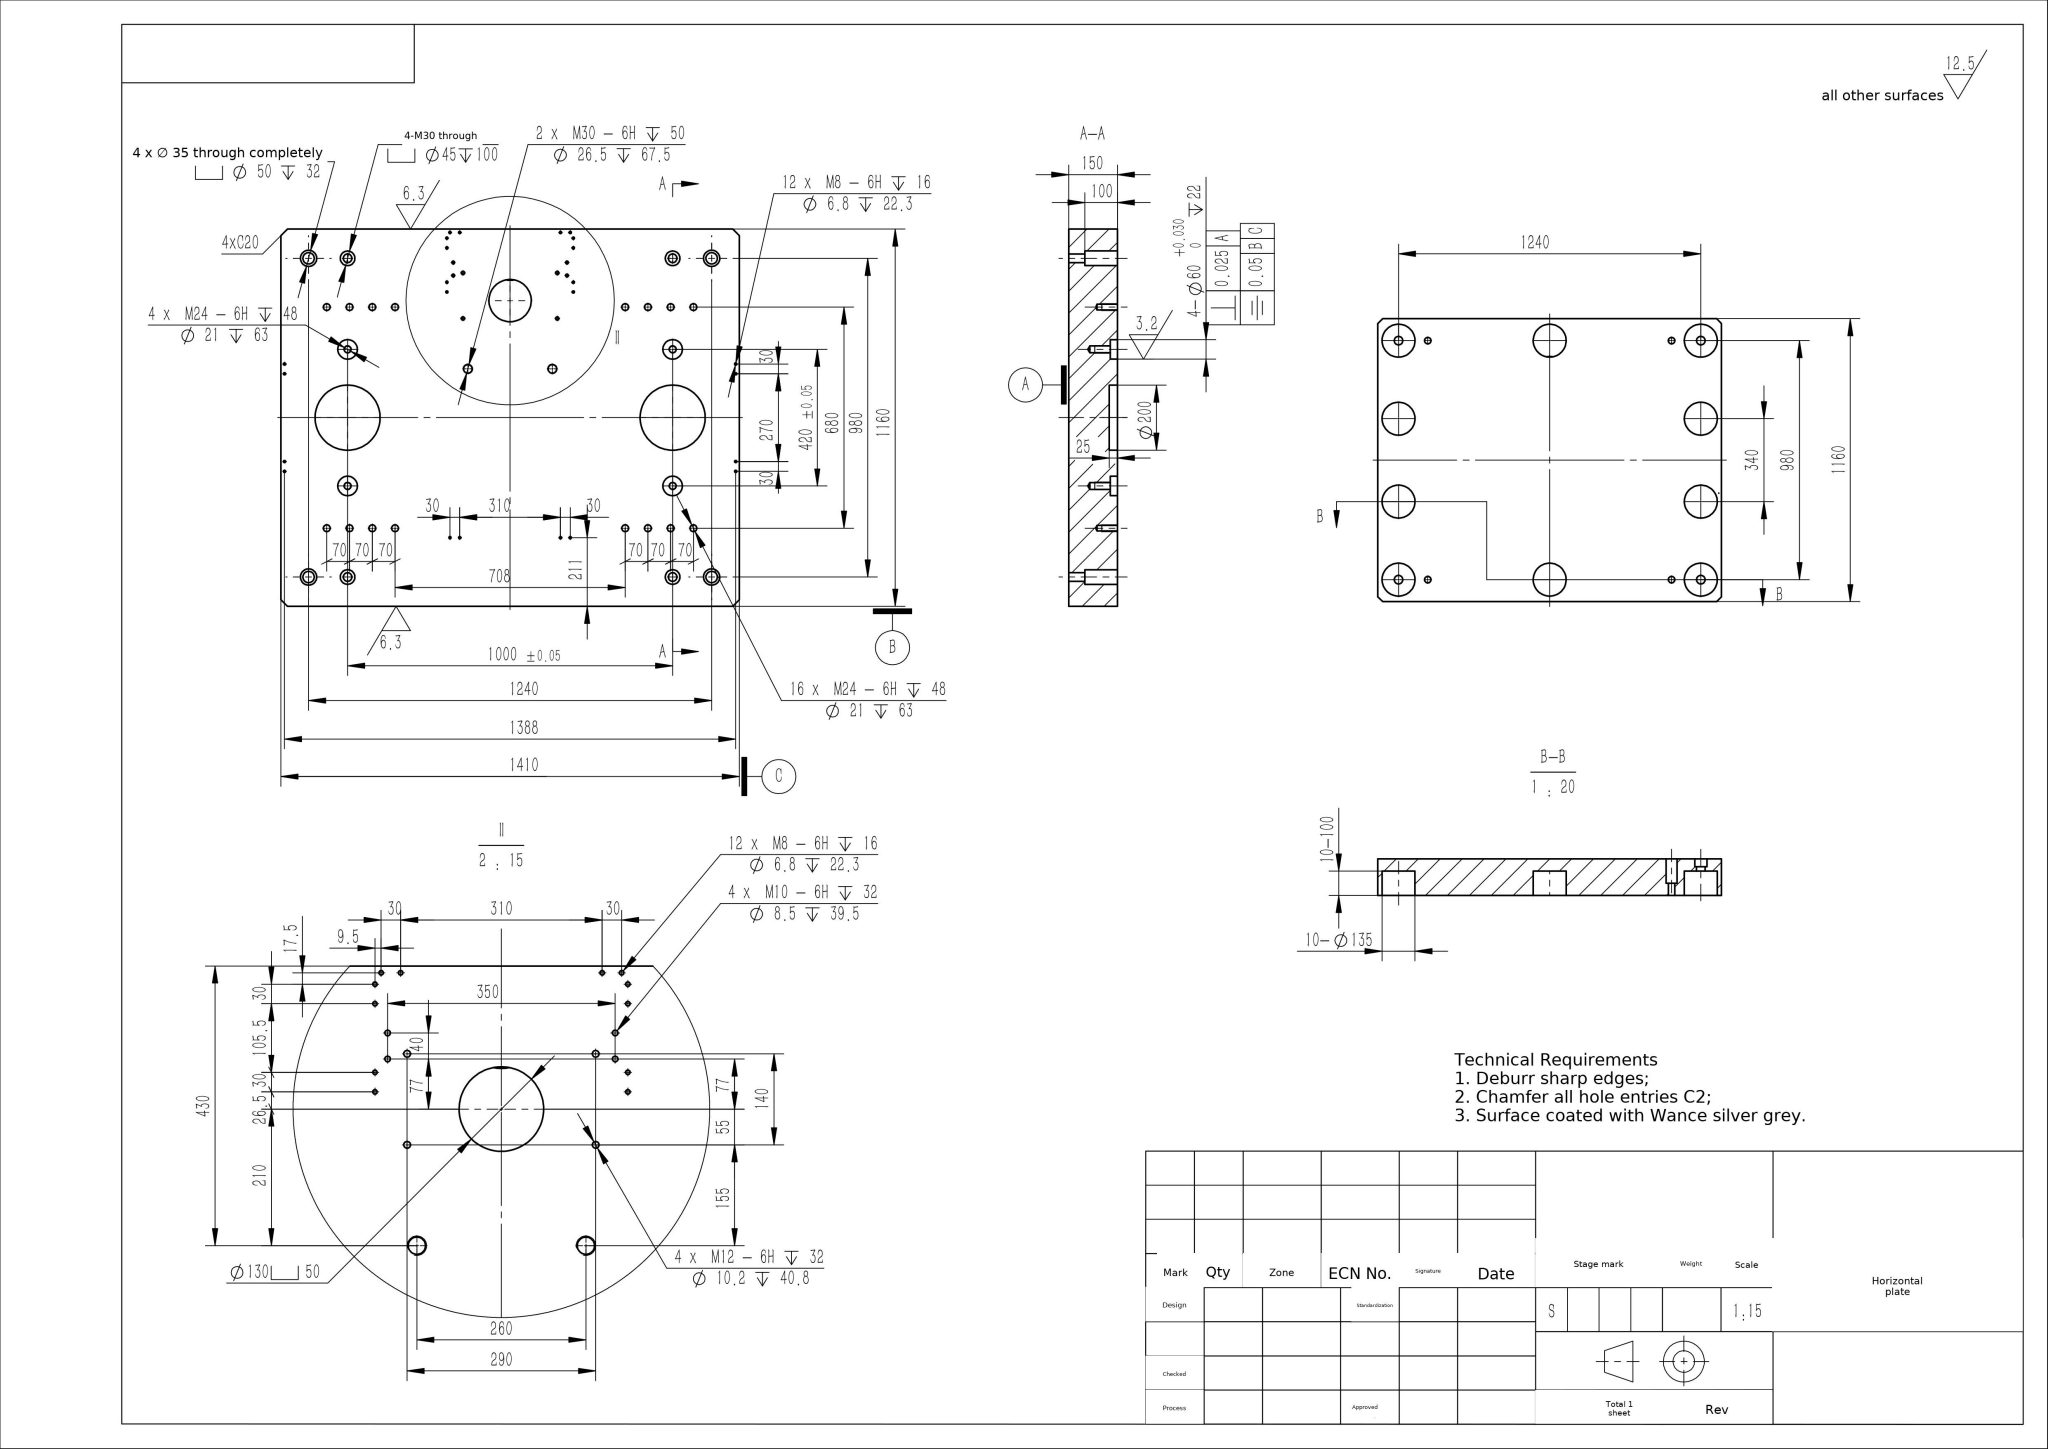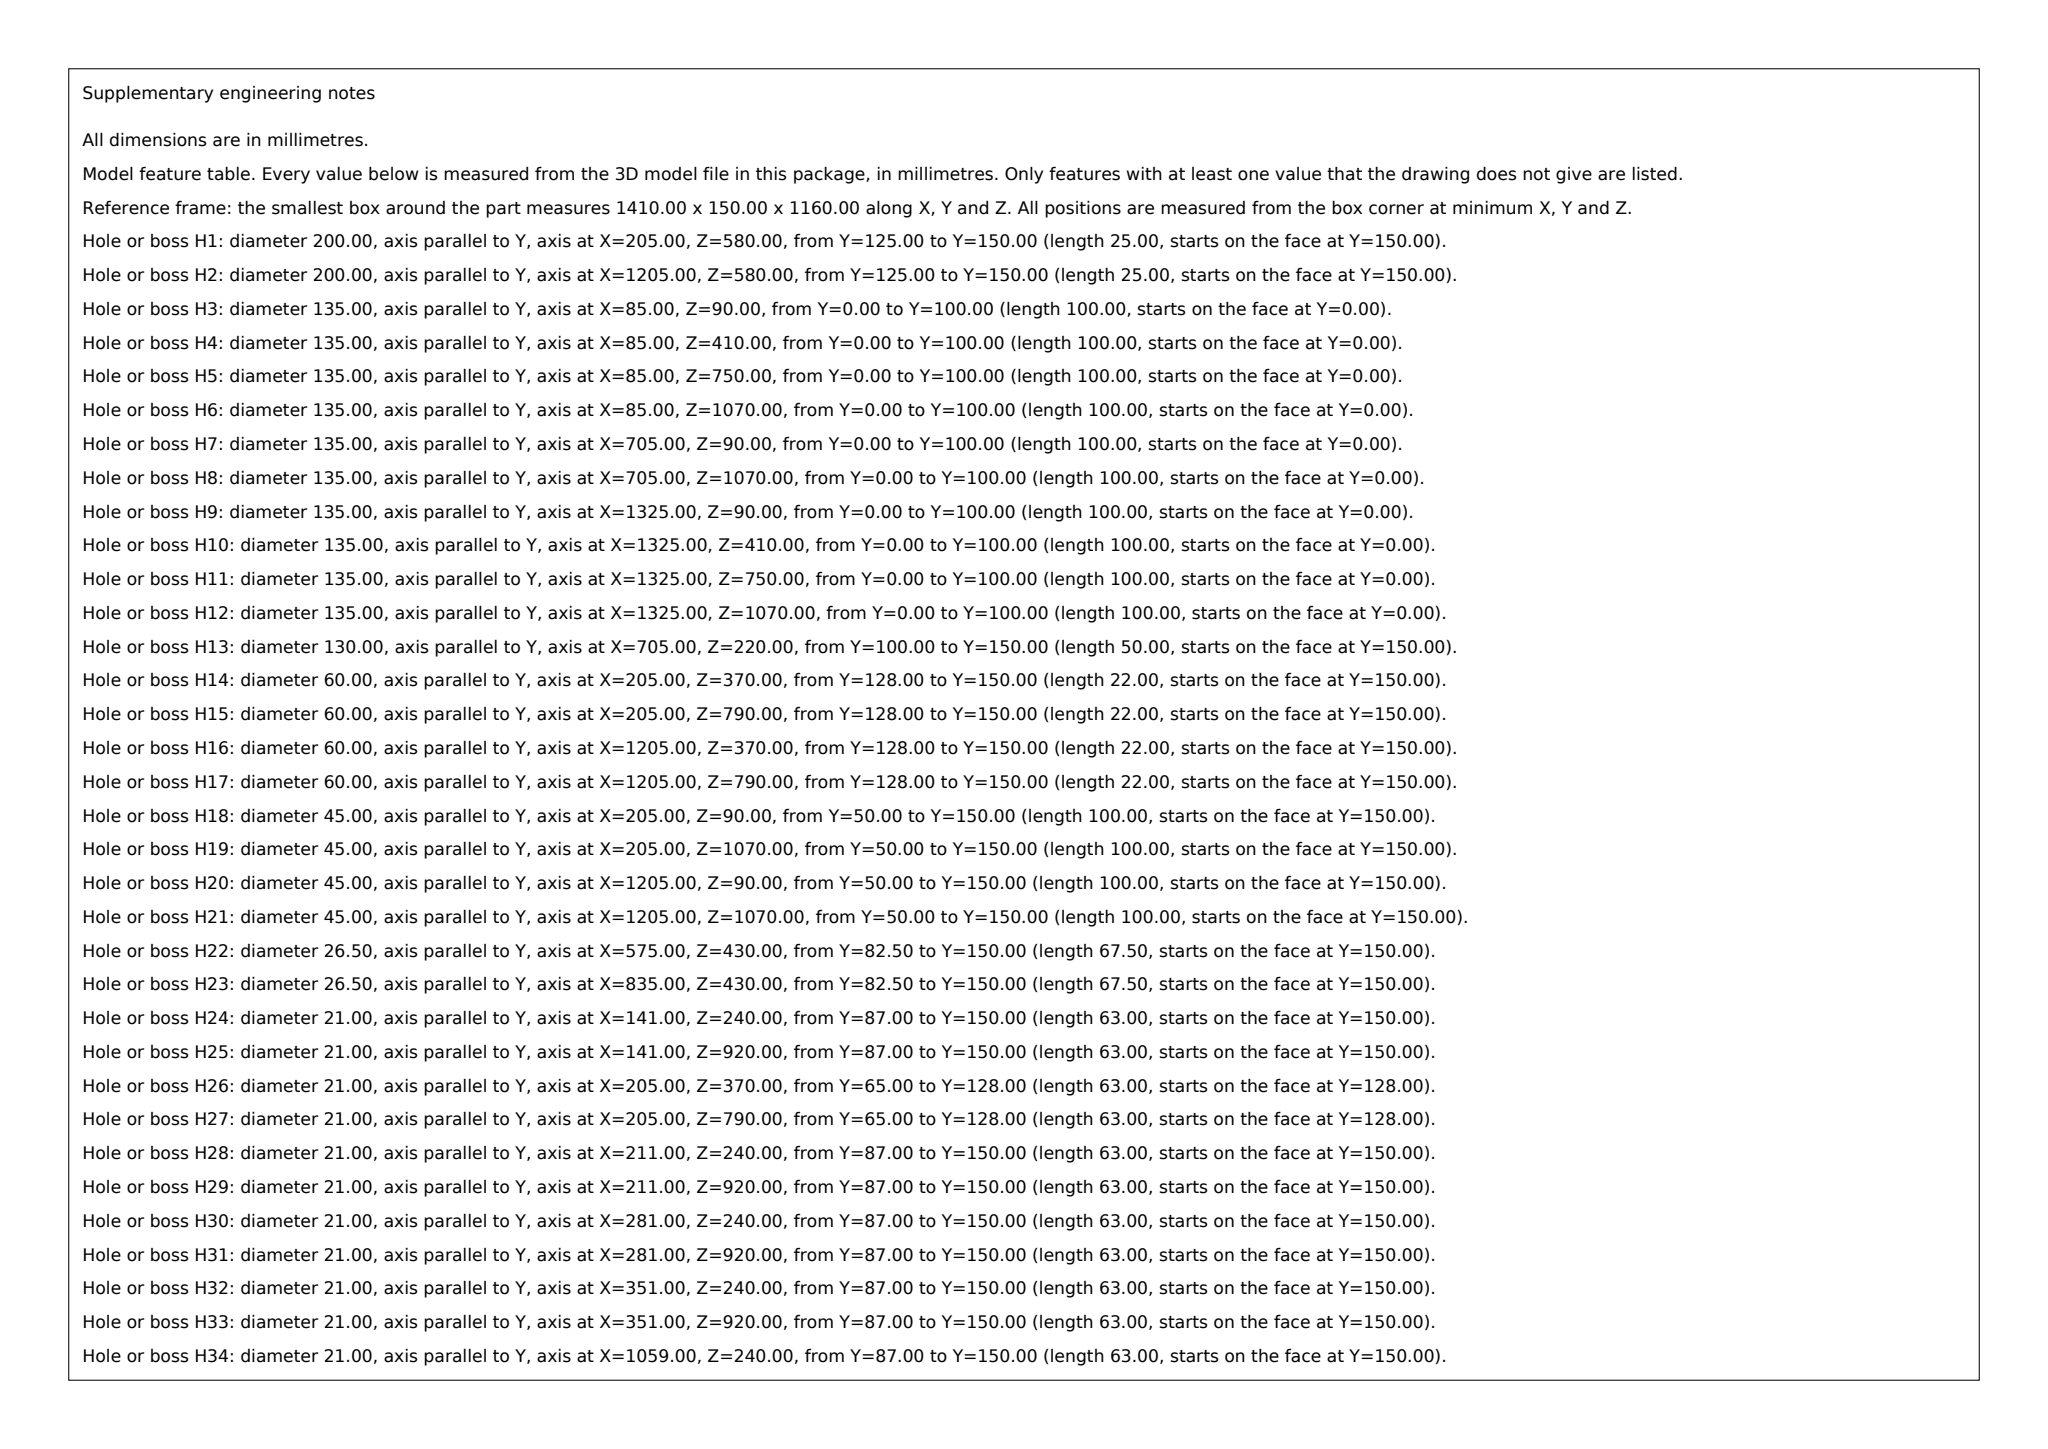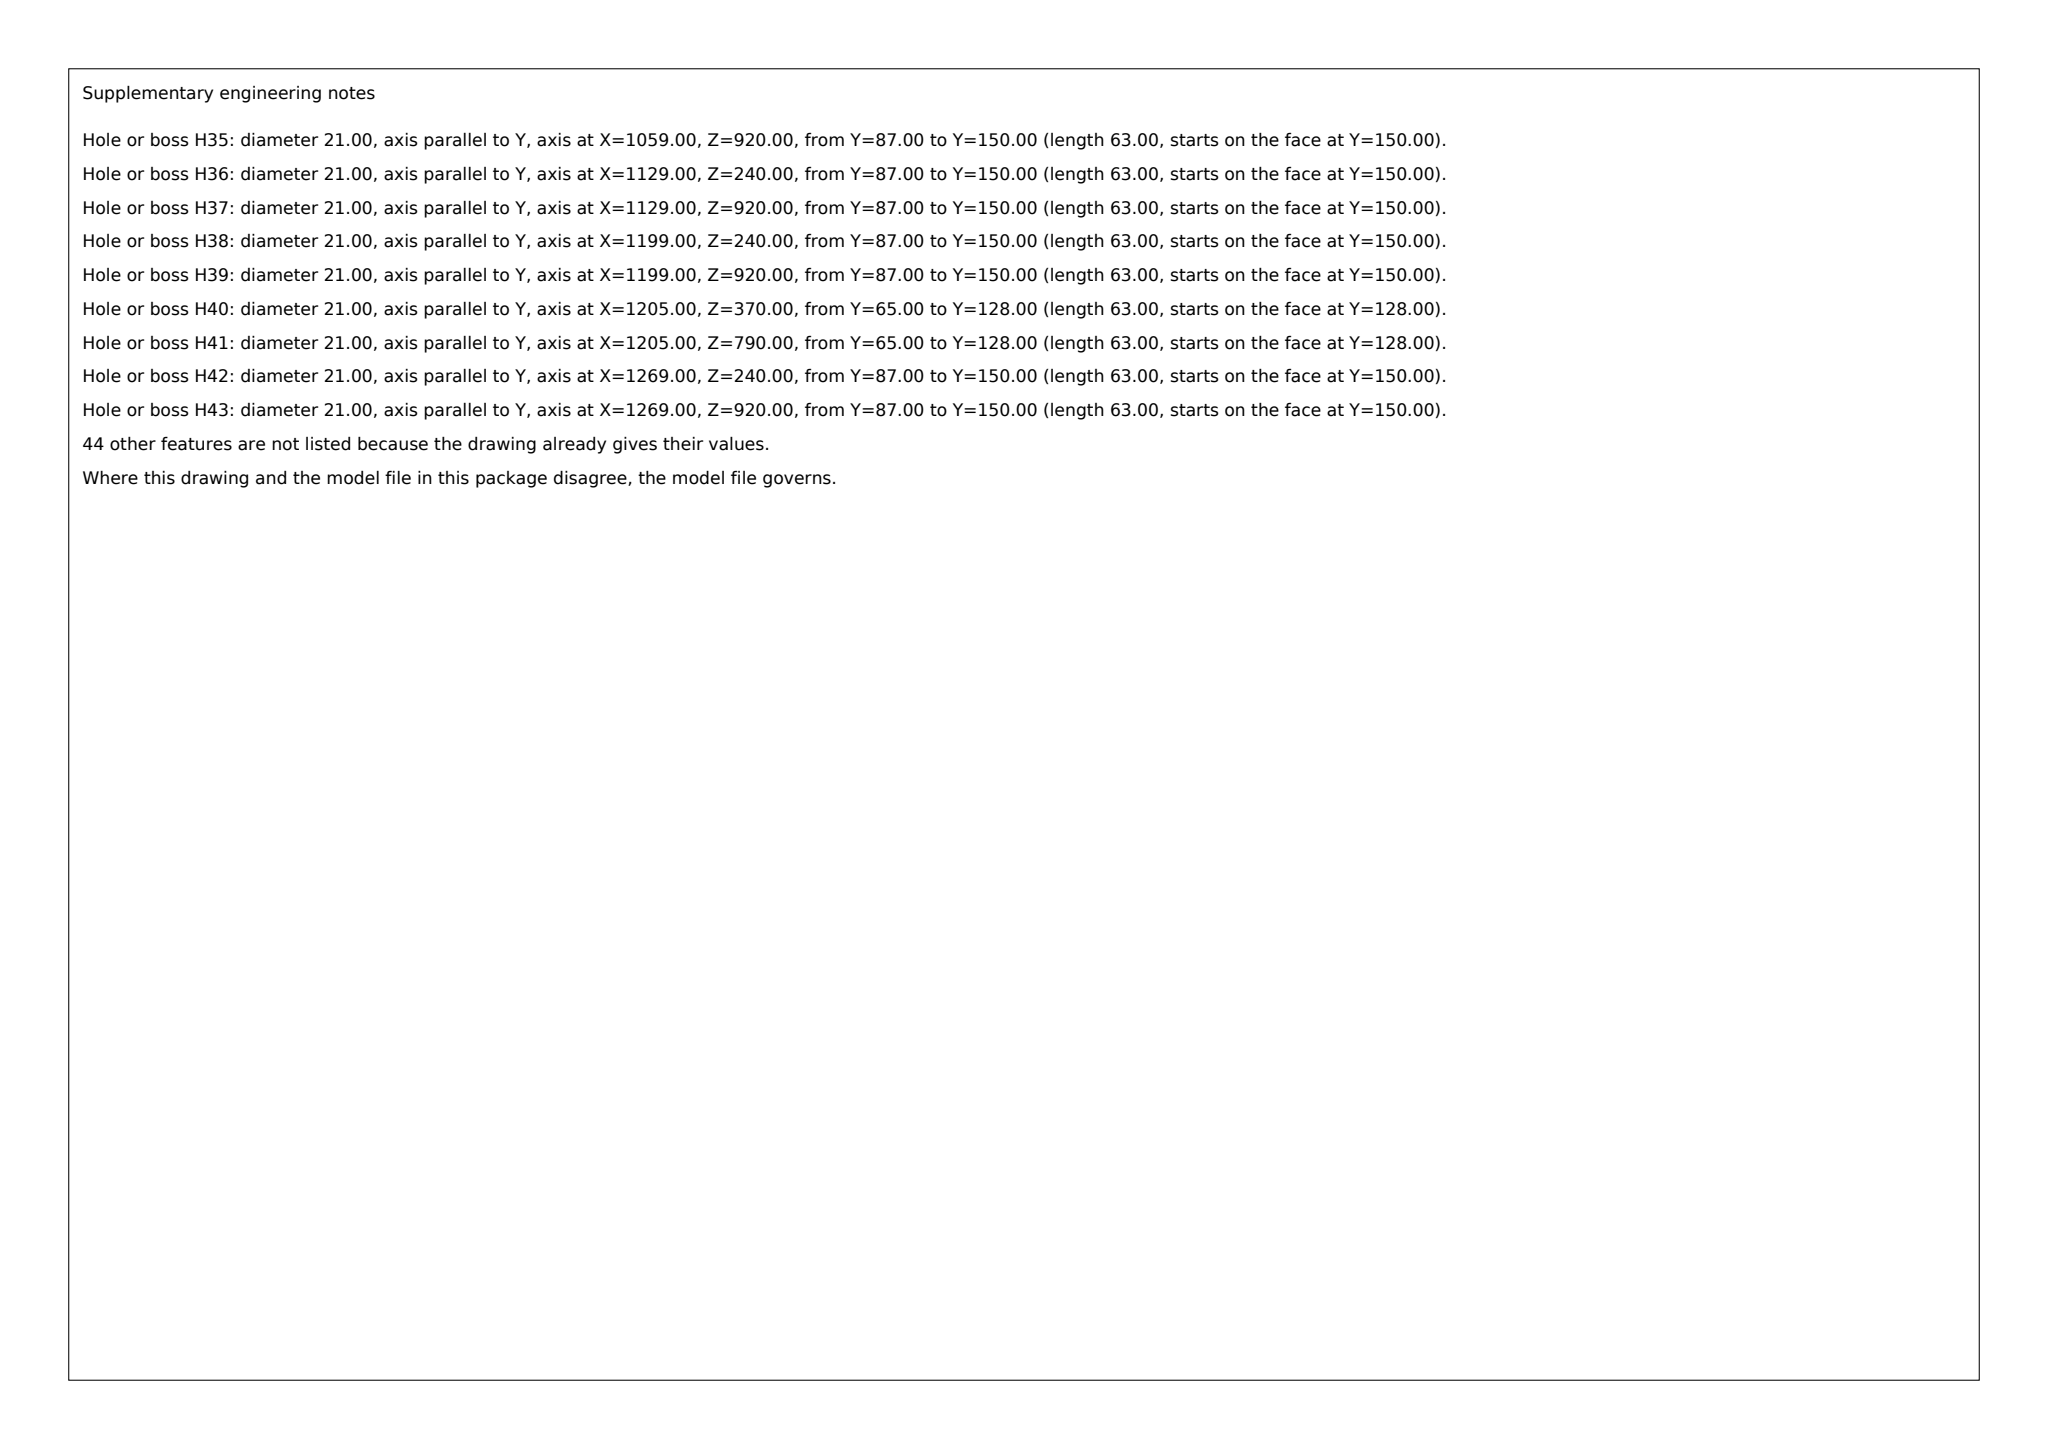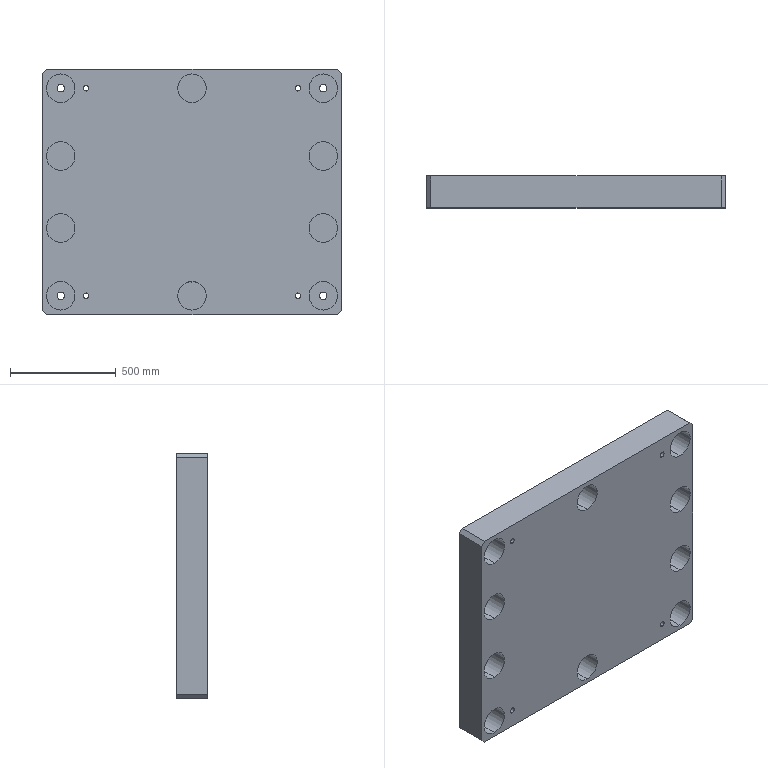Part | SolidWorks | mm | 1 solid | 317 faces | box 1410 x 150 x 1160 mm | volume 226784598 mm3 | cylinder 174 | cone 108 | plane 35 | commonest cylinder face diameters 6.8 x48 21 x40 135 x20 26.5 x12 45 x8 50 x8 35 x8 8.5 x8
build123d program:
from build123d import *

# Parameters (mm, degrees)
SKETCH2_W                                          = 1410
SKETCH2_H                                          = 720
BOSS_EXTRUDE1_DEPTH                                = 150
SKETCH4_R                                          = 100
CUT_EXTRUDE1_DEPTH                                 = 25
SKETCH6_R                                          = 30
CUT_EXTRUDE3_DEPTH                                 = 22
SKETCH24_W                                         = 1410
SKETCH24_H                                         = 150
BOSS_EXTRUDE5_DEPTH                                = 220
M12_TAPPED_HOLE1_D                                 = 10.2
M12_TAPPED_HOLE1_DEPTH                             = 40.75
M12_TAPPED_HOLE1_TIP                               = 3.064
SKETCH28_R                                         = 65
CUT_EXTRUDE8_DEPTH                                 = 50
SKETCH41_W                                         = 1410
SKETCH41_H                                         = 150
CUT_EXTRUDE11_DEPTH                                = 1
M30_TAPPED_HOLE1_D                                 = 26.5
M30_TAPPED_HOLE1_DEPTH                             = 67.5
M30_TAPPED_HOLE1_TIP                               = 7.961
M10_TAPPED_HOLE2_D                                 = 8.5
M10_TAPPED_HOLE2_DEPTH                             = 39.5
M10_TAPPED_HOLE2_TIP                               = 2.554
SKETCH60_W                                         = 1410
SKETCH60_H                                         = 150
BOSS_EXTRUDE7_DEPTH                                = 24
SKETCH67_W                                         = 1410
SKETCH67_H                                         = 150
BOSS_EXTRUDE9_DEPTH                                = 197
M24_TAPPED_HOLE1_AT_2_COUNT                        = 2
M24_TAPPED_HOLE1_AT_2_PITCH                        = 70
M24_TAPPED_HOLE1_AT_3_COUNT                        = 2
M24_TAPPED_HOLE1_AT_3_PITCH                        = 140
M24_TAPPED_HOLE1_AT_4_COUNT                        = 2
M24_TAPPED_HOLE1_AT_4_PITCH                        = 210
SKETCH73_R                                         = 67.5
CUT_EXTRUDE15_DEPTH                                = 100
HOLE_SIZE_ACCORDING_TO_TYPE_1_OF_HEXAG_D           = 35
HOLE_SIZE_ACCORDING_TO_TYPE_1_OF_HEXAG_CBORE_D     = 50
HOLE_SIZE_ACCORDING_TO_TYPE_1_OF_HEXAG_CBORE_DEPTH = 32
HOLE_SIZE_ACCORDING_TO_TYPE_1_OF_H_2_D             = 35
HOLE_SIZE_ACCORDING_TO_TYPE_1_OF_H_2_CBORE_D       = 50
HOLE_SIZE_ACCORDING_TO_TYPE_1_OF_H_2_CBORE_DEPTH   = 32
M30_TAPPED_HOLE2_D                                 = 26.5
SKETCH77_R                                         = 22.5
CUT_EXTRUDE16_DEPTH                                = 100
M8_TAPPED_HOLE1_D                                  = 6.8
M8_TAPPED_HOLE1_DEPTH                              = 22.25
M8_TAPPED_HOLE1_TIP                                = 2.043
M24_TAPPED_HOLE2_D                                 = 21
M24_TAPPED_HOLE2_DEPTH                             = 63
M24_TAPPED_HOLE2_TIP                               = 6.309
CHAMFER1_SIZE                                      = 20


with BuildPart() as part:
    # Sketch2 → Boss-Extrude1 (new body)
    with BuildSketch(Plane(origin=(0, 0, 0), x_dir=(1, 0, 0), z_dir=(0, 1, 0))):
        Rectangle(SKETCH2_W, SKETCH2_H)
    extrude(amount=-BOSS_EXTRUDE1_DEPTH)

    # Sketch4 → Cut-Extrude1 (cut)
    with BuildSketch(Plane(origin=(0, 0, 0), x_dir=(-1, 0, 0), z_dir=(0, 1, 0))):
        with Locations(Location((-500, 0, 0), (0, 0, 90))):
            Circle(SKETCH4_R)
        with Locations(Location((500, 0, 0), (0, 0, 90))):
            Circle(SKETCH4_R)
    extrude(amount=-CUT_EXTRUDE1_DEPTH, mode=Mode.SUBTRACT)

    # Sketch6 → Cut-Extrude3 (cut)
    with BuildSketch(Plane(origin=(0, 0, 0), x_dir=(-1, 0, 0), z_dir=(0, 1, 0))):
        with Locations(Location((-500, 210, 0), (0, 0, 90))):
            Circle(SKETCH6_R)
        with Locations(Location((500, 210, 0), (0, 0, 90))):
            Circle(SKETCH6_R)
        with Locations(Location((500, -210, 0), (0, 0, 90))):
            Circle(SKETCH6_R)
        with Locations(Location((-500, -210, 0), (0, 0, 90))):
            Circle(SKETCH6_R)
    extrude(amount=-CUT_EXTRUDE3_DEPTH, mode=Mode.SUBTRACT)

    # Sketch24 → Boss-Extrude5 (add)
    with BuildSketch(Plane(origin=(0, 0, -360), x_dir=(-1, 0, 0), z_dir=(0, 0, -1))):
        with Locations((0, -75)):
            Rectangle(SKETCH24_W, SKETCH24_H)
    extrude(amount=BOSS_EXTRUDE5_DEPTH)

    # M12 Tapped Hole1
    with Locations(Plane(origin=(0, 0, 0), x_dir=(1, 0, 0), z_dir=(0, 1, 0))):
        with Locations((145, 305), (145, 445), (-145, 305), (-145, 445)):
            Hole(M12_TAPPED_HOLE1_D / 2, depth=M12_TAPPED_HOLE1_DEPTH)
            with Locations((0, 0, -(M12_TAPPED_HOLE1_DEPTH + M12_TAPPED_HOLE1_TIP / 2))):  # 118° drill point
                Cone(0, M12_TAPPED_HOLE1_D / 2, M12_TAPPED_HOLE1_TIP, mode=Mode.SUBTRACT)

    # Sketch28 → Cut-Extrude8 (cut)
    with BuildSketch(Plane(origin=(0, 0, 0), x_dir=(-1, 0, 0), z_dir=(0, 1, 0))):
        with Locations(Location((0, -360, 0), (0, 0, 90))):
            Circle(SKETCH28_R)
    extrude(amount=-CUT_EXTRUDE8_DEPTH, mode=Mode.SUBTRACT)

    # Sketch41 → Cut-Extrude11 (cut)
    with BuildSketch(Plane.XY.offset(360)):
        with Locations((0, -75)):
            Rectangle(SKETCH41_W, SKETCH41_H)
    extrude(amount=-CUT_EXTRUDE11_DEPTH, mode=Mode.SUBTRACT)

    # M30 Tapped Hole1
    with Locations(Plane(origin=(0, 0, 0), x_dir=(1, 0, 0), z_dir=(0, 1, 0))):
        with Locations((130, 150), (-130, 150)):
            Hole(M30_TAPPED_HOLE1_D / 2, depth=M30_TAPPED_HOLE1_DEPTH)
            with Locations((0, 0, -(M30_TAPPED_HOLE1_DEPTH + M30_TAPPED_HOLE1_TIP / 2))):  # 118° drill point
                Cone(0, M30_TAPPED_HOLE1_D / 2, M30_TAPPED_HOLE1_TIP, mode=Mode.SUBTRACT)

    # M10 Tapped Hole2
    with Locations(Plane(origin=(0, 0, 0), x_dir=(1, 0, 0), z_dir=(0, 1, 0))):
        with Locations((175, 477), (175, 437), (-175, 477), (-175, 437)):
            Hole(M10_TAPPED_HOLE2_D / 2, depth=M10_TAPPED_HOLE2_DEPTH)
            with Locations((0, 0, -(M10_TAPPED_HOLE2_DEPTH + M10_TAPPED_HOLE2_TIP / 2))):  # 118° drill point
                Cone(0, M10_TAPPED_HOLE2_D / 2, M10_TAPPED_HOLE2_TIP, mode=Mode.SUBTRACT)

    # Sketch60 → Boss-Extrude7 (add)
    with BuildSketch(Plane.XY.offset(359)):
        with Locations((0, -75)):
            Rectangle(SKETCH60_W, SKETCH60_H)
    extrude(amount=BOSS_EXTRUDE7_DEPTH)

    # Sketch67 → Boss-Extrude9 (add)
    with BuildSketch(Plane.XY.offset(383)):
        with Locations((0, -75)):
            Rectangle(SKETCH67_W, SKETCH67_H)
    extrude(amount=BOSS_EXTRUDE9_DEPTH)

    # Sketch71 → M24 Tapped Hole1 (revolve, cut)
    with BuildSketch(Plane(origin=(354, 0, -340), x_dir=(0, 0, 1), z_dir=(1, 0, 0))):
        Polygon((0, 0), (0, 69.309), (10.5, 63), (10.5, 0), align=None)
    m24_tapped_hole1 = revolve(axis=Axis((354, 6.35, -340), (0, -1, 0)), mode=Mode.SUBTRACT)

    # M24 Tapped Hole1 at 2: M24 Tapped Hole1 ×2
    with Locations(*[(i * M24_TAPPED_HOLE1_AT_2_PITCH, 0, 0) for i in range(1, M24_TAPPED_HOLE1_AT_2_COUNT)]):
        add(m24_tapped_hole1, mode=Mode.SUBTRACT)

    # M24 Tapped Hole1 at 3: M24 Tapped Hole1 ×2
    with Locations(*[(i * M24_TAPPED_HOLE1_AT_3_PITCH, 0, 0) for i in range(1, M24_TAPPED_HOLE1_AT_3_COUNT)]):
        add(m24_tapped_hole1, mode=Mode.SUBTRACT)

    # M24 Tapped Hole1 at 4: M24 Tapped Hole1 ×2
    with Locations(*[(i * M24_TAPPED_HOLE1_AT_4_PITCH, 0, 0) for i in range(1, M24_TAPPED_HOLE1_AT_4_COUNT)]):
        add(m24_tapped_hole1, mode=Mode.SUBTRACT)

    # Mirror11: M24 Tapped Hole1 across plane
    add(m24_tapped_hole1.mirror(Plane(origin=(0, 0, 0), x_dir=(0, 0, 1), z_dir=(1, 0, 0))), mode=Mode.SUBTRACT)

    # Mirror11 copy 1 sketch → Mirror11 copy 1 (revolve, cut)
    with BuildSketch(Plane(origin=(-424, 0, -340), x_dir=(0, 0, 1), z_dir=(-1, 0, 0))):
        Polygon((0, 0), (0, -69.309), (10.5, -63), (10.5, 0), align=None)
    revolve(axis=Axis((-424, 6.35, -340), (0, 1, 0)), mode=Mode.SUBTRACT)

    # Mirror11 copy 2 sketch → Mirror11 copy 2 (revolve, cut)
    with BuildSketch(Plane(origin=(-494, 0, -340), x_dir=(0, 0, 1), z_dir=(-1, 0, 0))):
        Polygon((0, 0), (0, -69.309), (10.5, -63), (10.5, 0), align=None)
    revolve(axis=Axis((-494, 6.35, -340), (0, 1, 0)), mode=Mode.SUBTRACT)

    # Mirror11 copy 3 sketch → Mirror11 copy 3 (revolve, cut)
    with BuildSketch(Plane(origin=(-564, 0, -340), x_dir=(0, 0, 1), z_dir=(-1, 0, 0))):
        Polygon((0, 0), (0, -69.309), (10.5, -63), (10.5, 0), align=None)
    revolve(axis=Axis((-564, 6.35, -340), (0, 1, 0)), mode=Mode.SUBTRACT)

    # Mirror12: M24 Tapped Hole1 across plane
    add(m24_tapped_hole1.mirror(Plane.XY), mode=Mode.SUBTRACT)

    # Mirror12 copy 1 sketch → Mirror12 copy 1 (revolve, cut)
    with BuildSketch(Plane(origin=(424, 0, 340), x_dir=(0, 0, -1), z_dir=(1, 0, 0))):
        Polygon((0, 0), (0, -69.309), (10.5, -63), (10.5, 0), align=None)
    revolve(axis=Axis((424, 6.35, 340), (0, 1, 0)), mode=Mode.SUBTRACT)

    # Mirror12 copy 2 sketch → Mirror12 copy 2 (revolve, cut)
    with BuildSketch(Plane(origin=(494, 0, 340), x_dir=(0, 0, -1), z_dir=(1, 0, 0))):
        Polygon((0, 0), (0, -69.309), (10.5, -63), (10.5, 0), align=None)
    revolve(axis=Axis((494, 6.35, 340), (0, 1, 0)), mode=Mode.SUBTRACT)

    # Mirror12 copy 3 sketch → Mirror12 copy 3 (revolve, cut)
    with BuildSketch(Plane(origin=(564, 0, 340), x_dir=(0, 0, -1), z_dir=(1, 0, 0))):
        Polygon((0, 0), (0, -69.309), (10.5, -63), (10.5, 0), align=None)
    revolve(axis=Axis((564, 6.35, 340), (0, 1, 0)), mode=Mode.SUBTRACT)

    # Mirror12 copy 4 sketch → Mirror12 copy 4 (revolve, cut)
    with BuildSketch(Plane(origin=(-354, 0, 340), x_dir=(0, 0, -1), z_dir=(-1, 0, 0))):
        Polygon((0, 0), (0, 69.309), (10.5, 63), (10.5, 0), align=None)
    revolve(axis=Axis((-354, 6.35, 340), (0, -1, 0)), mode=Mode.SUBTRACT)

    # Mirror12 copy 5 sketch → Mirror12 copy 5 (revolve, cut)
    with BuildSketch(Plane(origin=(-424, 0, 340), x_dir=(0, 0, -1), z_dir=(-1, 0, 0))):
        Polygon((0, 0), (0, 69.309), (10.5, 63), (10.5, 0), align=None)
    revolve(axis=Axis((-424, 6.35, 340), (0, -1, 0)), mode=Mode.SUBTRACT)

    # Mirror12 copy 6 sketch → Mirror12 copy 6 (revolve, cut)
    with BuildSketch(Plane(origin=(-494, 0, 340), x_dir=(0, 0, -1), z_dir=(-1, 0, 0))):
        Polygon((0, 0), (0, 69.309), (10.5, 63), (10.5, 0), align=None)
    revolve(axis=Axis((-494, 6.35, 340), (0, -1, 0)), mode=Mode.SUBTRACT)

    # Mirror12 copy 7 sketch → Mirror12 copy 7 (revolve, cut)
    with BuildSketch(Plane(origin=(-564, 0, 340), x_dir=(0, 0, -1), z_dir=(-1, 0, 0))):
        Polygon((0, 0), (0, 69.309), (10.5, 63), (10.5, 0), align=None)
    revolve(axis=Axis((-564, 6.35, 340), (0, -1, 0)), mode=Mode.SUBTRACT)

    # Sketch73 → Cut-Extrude15 (cut)
    with BuildSketch(Plane(origin=(0, -150, 0), x_dir=(-1, 0, 0), z_dir=(0, -1, 0))):
        with Locations(Location((-620, 490, 0), (0, 0, 90))):
            Circle(SKETCH73_R)
        with Locations(Location((-620, -490, 0), (0, 0, 90))):
            Circle(SKETCH73_R)
        with Locations(Location((0, 490, 0), (0, 0, 90))):
            Circle(SKETCH73_R)
        with Locations(Location((620, 490, 0), (0, 0, 90))):
            Circle(SKETCH73_R)
        with Locations(Location((0, -490, 0), (0, 0, 90))):
            Circle(SKETCH73_R)
        with Locations(Location((620, -490, 0), (0, 0, 90))):
            Circle(SKETCH73_R)
        with Locations(Location((-620, 170, 0), (0, 0, 90))):
            Circle(SKETCH73_R)
        with Locations(Location((-620, -170, 0), (0, 0, 90))):
            Circle(SKETCH73_R)
        with Locations(Location((620, 170, 0), (0, 0, 270))):
            Circle(SKETCH73_R)
        with Locations(Location((620, -170, 0), (0, 0, 270))):
            Circle(SKETCH73_R)
    extrude(amount=-CUT_EXTRUDE15_DEPTH, mode=Mode.SUBTRACT)

    # Hole Size _According to_ Type 1 of Hexag (through all)
    with Locations(Plane(origin=(620, 0, 490), x_dir=(0, 0, 1), z_dir=(0, 1, 0))):
        with Locations((0, 0), (0, -1240), (-980, 0), (-980, -1240)):
            CounterBoreHole(HOLE_SIZE_ACCORDING_TO_TYPE_1_OF_HEXAG_D / 2, HOLE_SIZE_ACCORDING_TO_TYPE_1_OF_HEXAG_CBORE_D / 2, HOLE_SIZE_ACCORDING_TO_TYPE_1_OF_HEXAG_CBORE_DEPTH)

    # Hole Size _According to_ Type 1 of H 2 (through all)
    with Locations(Plane(origin=(953.357, 689.934, 0), x_dir=(0, 0, 1), z_dir=(0, 1, 0))):
        with Locations((0, 0)):
            CounterBoreHole(HOLE_SIZE_ACCORDING_TO_TYPE_1_OF_H_2_D / 2, HOLE_SIZE_ACCORDING_TO_TYPE_1_OF_H_2_CBORE_D / 2, HOLE_SIZE_ACCORDING_TO_TYPE_1_OF_H_2_CBORE_DEPTH)

    # M30 Tapped Hole2 (through all)
    with Locations(Plane(origin=(500, 0, 490), x_dir=(0, 0, 1), z_dir=(0, 1, 0))):
        with Locations((0, 0), (0, -1000), (-980, -1000), (-980, 0)):
            Hole(M30_TAPPED_HOLE2_D / 2)

    # Sketch77 → Cut-Extrude16 (cut)
    with BuildSketch(Plane(origin=(0, 0, 0), x_dir=(-1, 0, 0), z_dir=(0, 1, 0))):
        with Locations(Location((-500, 490, 0), (0, 0, 90))):
            Circle(SKETCH77_R)
        with Locations(Location((500, 490, 0), (0, 0, 90))):
            Circle(SKETCH77_R)
        with Locations(Location((-500, -490, 0), (0, 0, 90))):
            Circle(SKETCH77_R)
        with Locations(Location((500, -490, 0), (0, 0, 90))):
            Circle(SKETCH77_R)
    extrude(amount=-CUT_EXTRUDE16_DEPTH, mode=Mode.SUBTRACT)

    # M8 Tapped Hole1
    with Locations(Plane(origin=(694, 0, 165), x_dir=(0, 0, 1), z_dir=(0, 1, 0))):
        with Locations((0, 0), (-30, 0), (-300, 0), (-330, 0), (204, -509), (204, -539), (204, -849), (204, -879), (0, -1388), (-30, -1388), (-300, -1388), (-330, -1388), (-551.5, -888.5), (-581.5, -888.5), (-687, -888.5), (-717, -888.5), (-734.5, -849), (-734.5, -879), (-734.5, -539), (-734.5, -509), (-717, -499.5), (-687, -499.5), (-581.5, -499.5), (-551.5, -499.5)):
            Hole(M8_TAPPED_HOLE1_D / 2, depth=M8_TAPPED_HOLE1_DEPTH)
            with Locations((0, 0, -(M8_TAPPED_HOLE1_DEPTH + M8_TAPPED_HOLE1_TIP / 2))):  # 118° drill point
                Cone(0, M8_TAPPED_HOLE1_D / 2, M8_TAPPED_HOLE1_TIP, mode=Mode.SUBTRACT)

    # M24 Tapped Hole2
    with Locations(Plane(origin=(0, -22, 0), x_dir=(1, 0, 0), z_dir=(0, 1, 0))):
        with Locations((-500, 210), (-500, -210), (500, 210), (500, -210)):
            Hole(M24_TAPPED_HOLE2_D / 2, depth=M24_TAPPED_HOLE2_DEPTH)
            with Locations((0, 0, -(M24_TAPPED_HOLE2_DEPTH + M24_TAPPED_HOLE2_TIP / 2))):  # 118° drill point
                Cone(0, M24_TAPPED_HOLE2_D / 2, M24_TAPPED_HOLE2_TIP, mode=Mode.SUBTRACT)

    # Chamfer1
    chamfer1_edges = [part.edges().sort_by_distance(p)[0] for p in [
        (705, -75, 580),
        (-705, -75, 580),
        (-705, -75, -580),
        (705, -75, -580),
    ]]
    chamfer(chamfer1_edges, length=CHAMFER1_SIZE)


solid = part.part